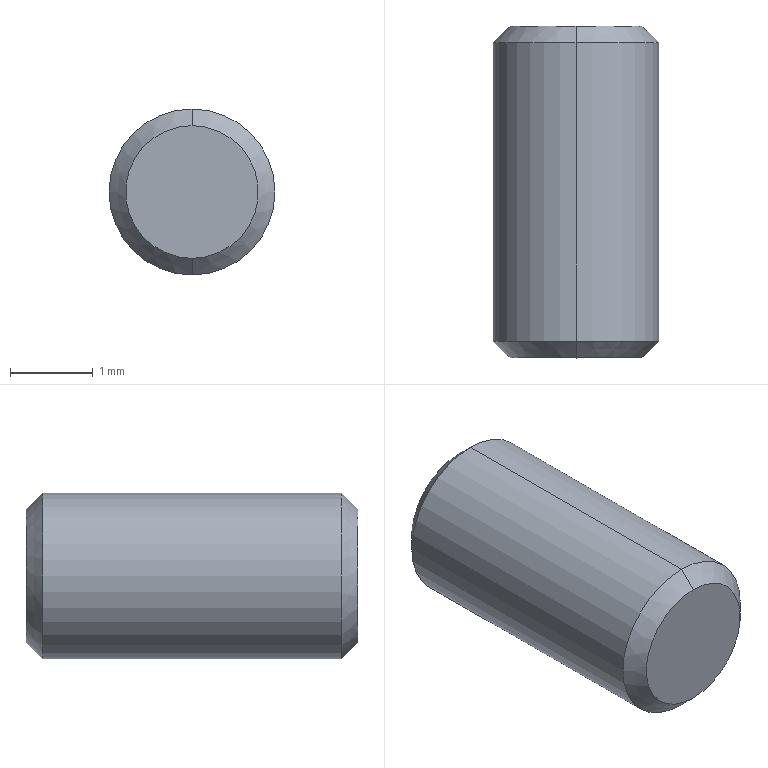Component | SolidWorks | BSH3-02-00ARubberBlankingAssembly2-1_BSH3-02-07Pin-1 | 1 solid | 8 faces | box 2 x 4 x 2 mm | volume 12 mm3 | cone 4 | cylinder 2 | plane 2 | commonest cylinder face diameters 2 x2
build123d program:
from build123d import *

# Parameters (mm, degrees)
SKETCH1_R      = 1
EXTRUDE1_DEPTH = 4
CHAMFER1_SIZE  = 0.2


with BuildPart() as part:
    # Sketch1 → Extrude1 (new body)
    with BuildSketch(Plane.XY):
        Circle(SKETCH1_R)
    extrude(amount=EXTRUDE1_DEPTH)

    # Chamfer1
    chamfer1_edges = [part.edges().sort_by_distance(p)[0] for p in [
        (-1, 0, 0),
        (-1, 0, 4),
    ]]
    chamfer(chamfer1_edges, length=CHAMFER1_SIZE)


solid = part.part

# Placed as in the assembly
solid = solid.moved(Location((102.629, 16.262, -2.239), (90, 0, 0)))
STEP:
#1=COLOUR_RGB('',0.7922,0.8196,0.9333);
#2=FILL_AREA_STYLE_COLOUR('',#1);
#3=FILL_AREA_STYLE('',(#2));
#4=SURFACE_STYLE_FILL_AREA(#3);
#5=SURFACE_SIDE_STYLE('',(#4));
#6=SURFACE_STYLE_USAGE(.BOTH.,#5);
#7=PRESENTATION_STYLE_ASSIGNMENT((#6));
#8=CARTESIAN_POINT('',(4.041,0.6402,-0.1197));
#9=VERTEX_POINT('',#8);
#10=CARTESIAN_POINT('',(4.041,0.6402,-0.05666));
#11=VERTEX_POINT('',#10);
#12=CARTESIAN_POINT('',(4.041,0.6402,-0.08816));
#13=DIRECTION('',(-0.,1.,-0.));
#14=DIRECTION('',(0.,0.,-1.));
#15=AXIS2_PLACEMENT_3D('',#12,#13,#14);
#16=CIRCLE('',#15,0.0315);
#17=EDGE_CURVE('',#9,#11,#16,.T.);
#18=ORIENTED_EDGE('',*,*,#17,.F.);
#19=CARTESIAN_POINT('',(4.041,0.6323,-0.1275));
#20=VERTEX_POINT('',#19);
#21=CARTESIAN_POINT('',(4.041,0.6402,-0.1197));
#22=DIRECTION('',(0.,-0.7071,-0.7071));
#23=VECTOR('',#22,39.37);
#24=LINE('',#21,#23);
#25=EDGE_CURVE('',#9,#20,#24,.T.);
#26=ORIENTED_EDGE('',*,*,#25,.T.);
#27=CARTESIAN_POINT('',(4.041,0.6323,-0.04879));
#28=VERTEX_POINT('',#27);
#29=CARTESIAN_POINT('',(4.041,0.6323,-0.08816));
#30=DIRECTION('',(0.,-1.,0.));
#31=DIRECTION('',(0.,0.,-1.));
#32=AXIS2_PLACEMENT_3D('',#29,#30,#31);
#33=CIRCLE('',#32,0.03937);
#34=EDGE_CURVE('',#28,#20,#33,.T.);
#35=ORIENTED_EDGE('',*,*,#34,.F.);
#36=CARTESIAN_POINT('',(4.041,0.6402,-0.05666));
#37=DIRECTION('',(0.,-0.7071,0.7071));
#38=VECTOR('',#37,39.37);
#39=LINE('',#36,#38);
#40=EDGE_CURVE('',#11,#28,#39,.T.);
#41=ORIENTED_EDGE('',*,*,#40,.F.);
#42=EDGE_LOOP('',(#18,#26,#35,#41));
#43=FACE_OUTER_BOUND('',#42,.T.);
#44=CARTESIAN_POINT('',(4.041,0.6402,-0.08816));
#45=DIRECTION('',(0.,-1.,0.));
#46=DIRECTION('',(0.,0.,1.));
#47=AXIS2_PLACEMENT_3D('',#44,#45,#46);
#48=CONICAL_SURFACE('',#47,0.0315,0.7854);
#49=ADVANCED_FACE('',(#43),#48,.T.);
#50=CARTESIAN_POINT('',(4.041,0.4827,-0.05666));
#51=VERTEX_POINT('',#50);
#52=CARTESIAN_POINT('',(4.041,0.4827,-0.1197));
#53=VERTEX_POINT('',#52);
#54=CARTESIAN_POINT('',(4.041,0.4827,-0.08816));
#55=DIRECTION('',(0.,-1.,0.));
#56=DIRECTION('',(0.,0.,-1.));
#57=AXIS2_PLACEMENT_3D('',#54,#55,#56);
#58=CIRCLE('',#57,0.0315);
#59=EDGE_CURVE('',#51,#53,#58,.T.);
#60=ORIENTED_EDGE('',*,*,#59,.F.);
#61=CARTESIAN_POINT('',(4.041,0.4906,-0.04879));
#62=VERTEX_POINT('',#61);
#63=CARTESIAN_POINT('',(4.041,0.4906,-0.04879));
#64=DIRECTION('',(-0.,0.7071,0.7071));
#65=VECTOR('',#64,39.37);
#66=LINE('',#63,#65);
#67=EDGE_CURVE('',#51,#62,#66,.T.);
#68=ORIENTED_EDGE('',*,*,#67,.T.);
#69=CARTESIAN_POINT('',(4.041,0.4906,-0.1275));
#70=VERTEX_POINT('',#69);
#71=CARTESIAN_POINT('',(4.041,0.4906,-0.08816));
#72=DIRECTION('',(-0.,1.,-0.));
#73=DIRECTION('',(0.,0.,-1.));
#74=AXIS2_PLACEMENT_3D('',#71,#72,#73);
#75=CIRCLE('',#74,0.03937);
#76=EDGE_CURVE('',#70,#62,#75,.T.);
#77=ORIENTED_EDGE('',*,*,#76,.F.);
#78=CARTESIAN_POINT('',(4.041,0.4906,-0.1275));
#79=DIRECTION('',(-0.,0.7071,-0.7071));
#80=VECTOR('',#79,39.37);
#81=LINE('',#78,#80);
#82=EDGE_CURVE('',#53,#70,#81,.T.);
#83=ORIENTED_EDGE('',*,*,#82,.F.);
#84=EDGE_LOOP('',(#60,#68,#77,#83));
#85=FACE_OUTER_BOUND('',#84,.T.);
#86=CARTESIAN_POINT('',(4.041,0.4906,-0.08816));
#87=DIRECTION('',(-0.,1.,-0.));
#88=DIRECTION('',(0.,0.,-1.));
#89=AXIS2_PLACEMENT_3D('',#86,#87,#88);
#90=CONICAL_SURFACE('',#89,0.03937,0.7854);
#91=ADVANCED_FACE('',(#85),#90,.T.);
#92=ORIENTED_EDGE('',*,*,#34,.T.);
#93=CARTESIAN_POINT('',(4.041,0.6402,-0.1275));
#94=DIRECTION('',(0.,-1.,0.));
#95=VECTOR('',#94,39.37);
#96=LINE('',#93,#95);
#97=EDGE_CURVE('',#20,#70,#96,.T.);
#98=ORIENTED_EDGE('',*,*,#97,.T.);
#99=ORIENTED_EDGE('',*,*,#76,.T.);
#100=CARTESIAN_POINT('',(4.041,0.6402,-0.04879));
#101=DIRECTION('',(0.,-1.,0.));
#102=VECTOR('',#101,39.37);
#103=LINE('',#100,#102);
#104=EDGE_CURVE('',#28,#62,#103,.T.);
#105=ORIENTED_EDGE('',*,*,#104,.F.);
#106=EDGE_LOOP('',(#92,#98,#99,#105));
#107=FACE_OUTER_BOUND('',#106,.T.);
#108=CARTESIAN_POINT('',(4.041,0.6402,-0.08816));
#109=DIRECTION('',(0.,-1.,0.));
#110=DIRECTION('',(0.,0.,1.));
#111=AXIS2_PLACEMENT_3D('',#108,#109,#110);
#112=CYLINDRICAL_SURFACE('',#111,0.03937);
#113=ADVANCED_FACE('',(#107),#112,.T.);
#114=ORIENTED_EDGE('',*,*,#97,.F.);
#115=CARTESIAN_POINT('',(4.041,0.6323,-0.08816));
#116=DIRECTION('',(0.,-1.,0.));
#117=DIRECTION('',(0.,0.,-1.));
#118=AXIS2_PLACEMENT_3D('',#115,#116,#117);
#119=CIRCLE('',#118,0.03937);
#120=EDGE_CURVE('',#20,#28,#119,.T.);
#121=ORIENTED_EDGE('',*,*,#120,.T.);
#122=ORIENTED_EDGE('',*,*,#104,.T.);
#123=CARTESIAN_POINT('',(4.041,0.4906,-0.08816));
#124=DIRECTION('',(-0.,1.,-0.));
#125=DIRECTION('',(0.,0.,-1.));
#126=AXIS2_PLACEMENT_3D('',#123,#124,#125);
#127=CIRCLE('',#126,0.03937);
#128=EDGE_CURVE('',#62,#70,#127,.T.);
#129=ORIENTED_EDGE('',*,*,#128,.T.);
#130=EDGE_LOOP('',(#114,#121,#122,#129));
#131=FACE_OUTER_BOUND('',#130,.T.);
#132=CARTESIAN_POINT('',(4.041,0.6402,-0.08816));
#133=DIRECTION('',(0.,-1.,0.));
#134=DIRECTION('',(0.,0.,1.));
#135=AXIS2_PLACEMENT_3D('',#132,#133,#134);
#136=CYLINDRICAL_SURFACE('',#135,0.03937);
#137=ADVANCED_FACE('',(#131),#136,.T.);
#138=CARTESIAN_POINT('',(4.041,0.6402,-0.08816));
#139=DIRECTION('',(-0.,1.,-0.));
#140=DIRECTION('',(0.,0.,-1.));
#141=AXIS2_PLACEMENT_3D('',#138,#139,#140);
#142=CIRCLE('',#141,0.0315);
#143=EDGE_CURVE('',#11,#9,#142,.T.);
#144=ORIENTED_EDGE('',*,*,#143,.T.);
#145=ORIENTED_EDGE('',*,*,#17,.T.);
#146=EDGE_LOOP('',(#144,#145));
#147=FACE_OUTER_BOUND('',#146,.T.);
#148=CARTESIAN_POINT('',(4.041,0.6402,-0.08816));
#149=DIRECTION('',(-0.,1.,-0.));
#150=DIRECTION('',(-0.,-0.,-1.));
#151=AXIS2_PLACEMENT_3D('',#148,#149,#150);
#152=PLANE('',#151);
#153=ADVANCED_FACE('',(#147),#152,.T.);
#154=CARTESIAN_POINT('',(4.041,0.4827,-0.08816));
#155=DIRECTION('',(0.,-1.,0.));
#156=DIRECTION('',(0.,0.,-1.));
#157=AXIS2_PLACEMENT_3D('',#154,#155,#156);
#158=CIRCLE('',#157,0.0315);
#159=EDGE_CURVE('',#53,#51,#158,.T.);
#160=ORIENTED_EDGE('',*,*,#159,.T.);
#161=ORIENTED_EDGE('',*,*,#59,.T.);
#162=EDGE_LOOP('',(#160,#161));
#163=FACE_OUTER_BOUND('',#162,.T.);
#164=CARTESIAN_POINT('',(4.041,0.4827,-0.08816));
#165=DIRECTION('',(-0.,1.,-0.));
#166=DIRECTION('',(-0.,-0.,-1.));
#167=AXIS2_PLACEMENT_3D('',#164,#165,#166);
#168=PLANE('',#167);
#169=ADVANCED_FACE('',(#163),#168,.F.);
#170=ORIENTED_EDGE('',*,*,#67,.F.);
#171=ORIENTED_EDGE('',*,*,#159,.F.);
#172=ORIENTED_EDGE('',*,*,#82,.T.);
#173=ORIENTED_EDGE('',*,*,#128,.F.);
#174=EDGE_LOOP('',(#170,#171,#172,#173));
#175=FACE_OUTER_BOUND('',#174,.T.);
#176=CARTESIAN_POINT('',(4.041,0.4906,-0.08816));
#177=DIRECTION('',(-0.,1.,-0.));
#178=DIRECTION('',(0.,0.,-1.));
#179=AXIS2_PLACEMENT_3D('',#176,#177,#178);
#180=CONICAL_SURFACE('',#179,0.03937,0.7854);
#181=ADVANCED_FACE('',(#175),#180,.T.);
#182=ORIENTED_EDGE('',*,*,#25,.F.);
#183=ORIENTED_EDGE('',*,*,#143,.F.);
#184=ORIENTED_EDGE('',*,*,#40,.T.);
#185=ORIENTED_EDGE('',*,*,#120,.F.);
#186=EDGE_LOOP('',(#182,#183,#184,#185));
#187=FACE_OUTER_BOUND('',#186,.T.);
#188=CARTESIAN_POINT('',(4.041,0.6402,-0.08816));
#189=DIRECTION('',(0.,-1.,0.));
#190=DIRECTION('',(0.,0.,1.));
#191=AXIS2_PLACEMENT_3D('',#188,#189,#190);
#192=CONICAL_SURFACE('',#191,0.0315,0.7854);
#193=ADVANCED_FACE('',(#187),#192,.T.);
#194=CLOSED_SHELL('',(#49,#91,#113,#137,#153,#169,#181,#193));
#195=MANIFOLD_SOLID_BREP('',#194);
#196=STYLED_ITEM('',(#7),#195);
#197=(LENGTH_UNIT()NAMED_UNIT(*)SI_UNIT($,.METRE.));
#198=LENGTH_MEASURE_WITH_UNIT(LENGTH_MEASURE(0.0254),#197);
#199=DIMENSIONAL_EXPONENTS(1.,0.,0.,0.,0.,0.,0.);
#200=(CONVERSION_BASED_UNIT('',#198)LENGTH_UNIT()NAMED_UNIT(#199));
#201=UNCERTAINTY_MEASURE_WITH_UNIT(LENGTH_MEASURE(0.00001),#200,'','');
#202=(NAMED_UNIT(*)PLANE_ANGLE_UNIT()SI_UNIT($,.RADIAN.));
#203=(NAMED_UNIT(*)SI_UNIT($,.STERADIAN.)SOLID_ANGLE_UNIT());
#204=(GEOMETRIC_REPRESENTATION_CONTEXT(3)GLOBAL_UNCERTAINTY_ASSIGNED_CONTEXT((#201))GLOBAL_UNIT_ASSIGNED_CONTEXT((#200,#202,#203))REPRESENTATION_CONTEXT('',''));
#205=MECHANICAL_DESIGN_GEOMETRIC_PRESENTATION_REPRESENTATION('',(#196),#204);
#206=PRESENTATION_LAYER_ASSIGNMENT('','',(#196));
#207=CARTESIAN_POINT('',(0.,0.,0.));
#208=DIRECTION('',(0.,0.,1.));
#209=DIRECTION('',(1.,0.,0.));
#210=AXIS2_PLACEMENT_3D('',#207,#208,#209);
#211=(LENGTH_UNIT()NAMED_UNIT(*)SI_UNIT($,.METRE.));
#212=LENGTH_MEASURE_WITH_UNIT(LENGTH_MEASURE(0.0254),#211);
#213=DIMENSIONAL_EXPONENTS(1.,0.,0.,0.,0.,0.,0.);
#214=(CONVERSION_BASED_UNIT('',#212)LENGTH_UNIT()NAMED_UNIT(#213));
#215=UNCERTAINTY_MEASURE_WITH_UNIT(LENGTH_MEASURE(0.00001),#214,'','');
#216=(NAMED_UNIT(*)PLANE_ANGLE_UNIT()SI_UNIT($,.RADIAN.));
#217=(NAMED_UNIT(*)SI_UNIT($,.STERADIAN.)SOLID_ANGLE_UNIT());
#218=(GEOMETRIC_REPRESENTATION_CONTEXT(3)GLOBAL_UNCERTAINTY_ASSIGNED_CONTEXT((#215))GLOBAL_UNIT_ASSIGNED_CONTEXT((#214,#216,#217))REPRESENTATION_CONTEXT('',''));
#219=ADVANCED_BREP_SHAPE_REPRESENTATION('',(#195,#210),#218);